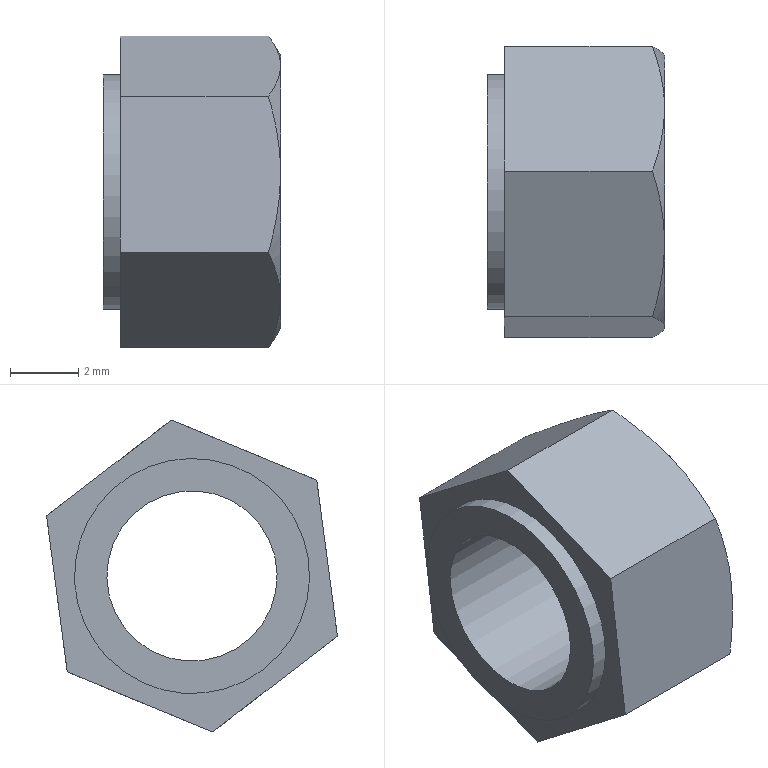Component | NX | GB-T6170_T-2000_M5X0_8 | 1 solid | 18 faces | volume 174 mm3 | plane 9 | cone 7 | cylinder 2 | commonest cylinder face diameters 6.9 x1 5 x1